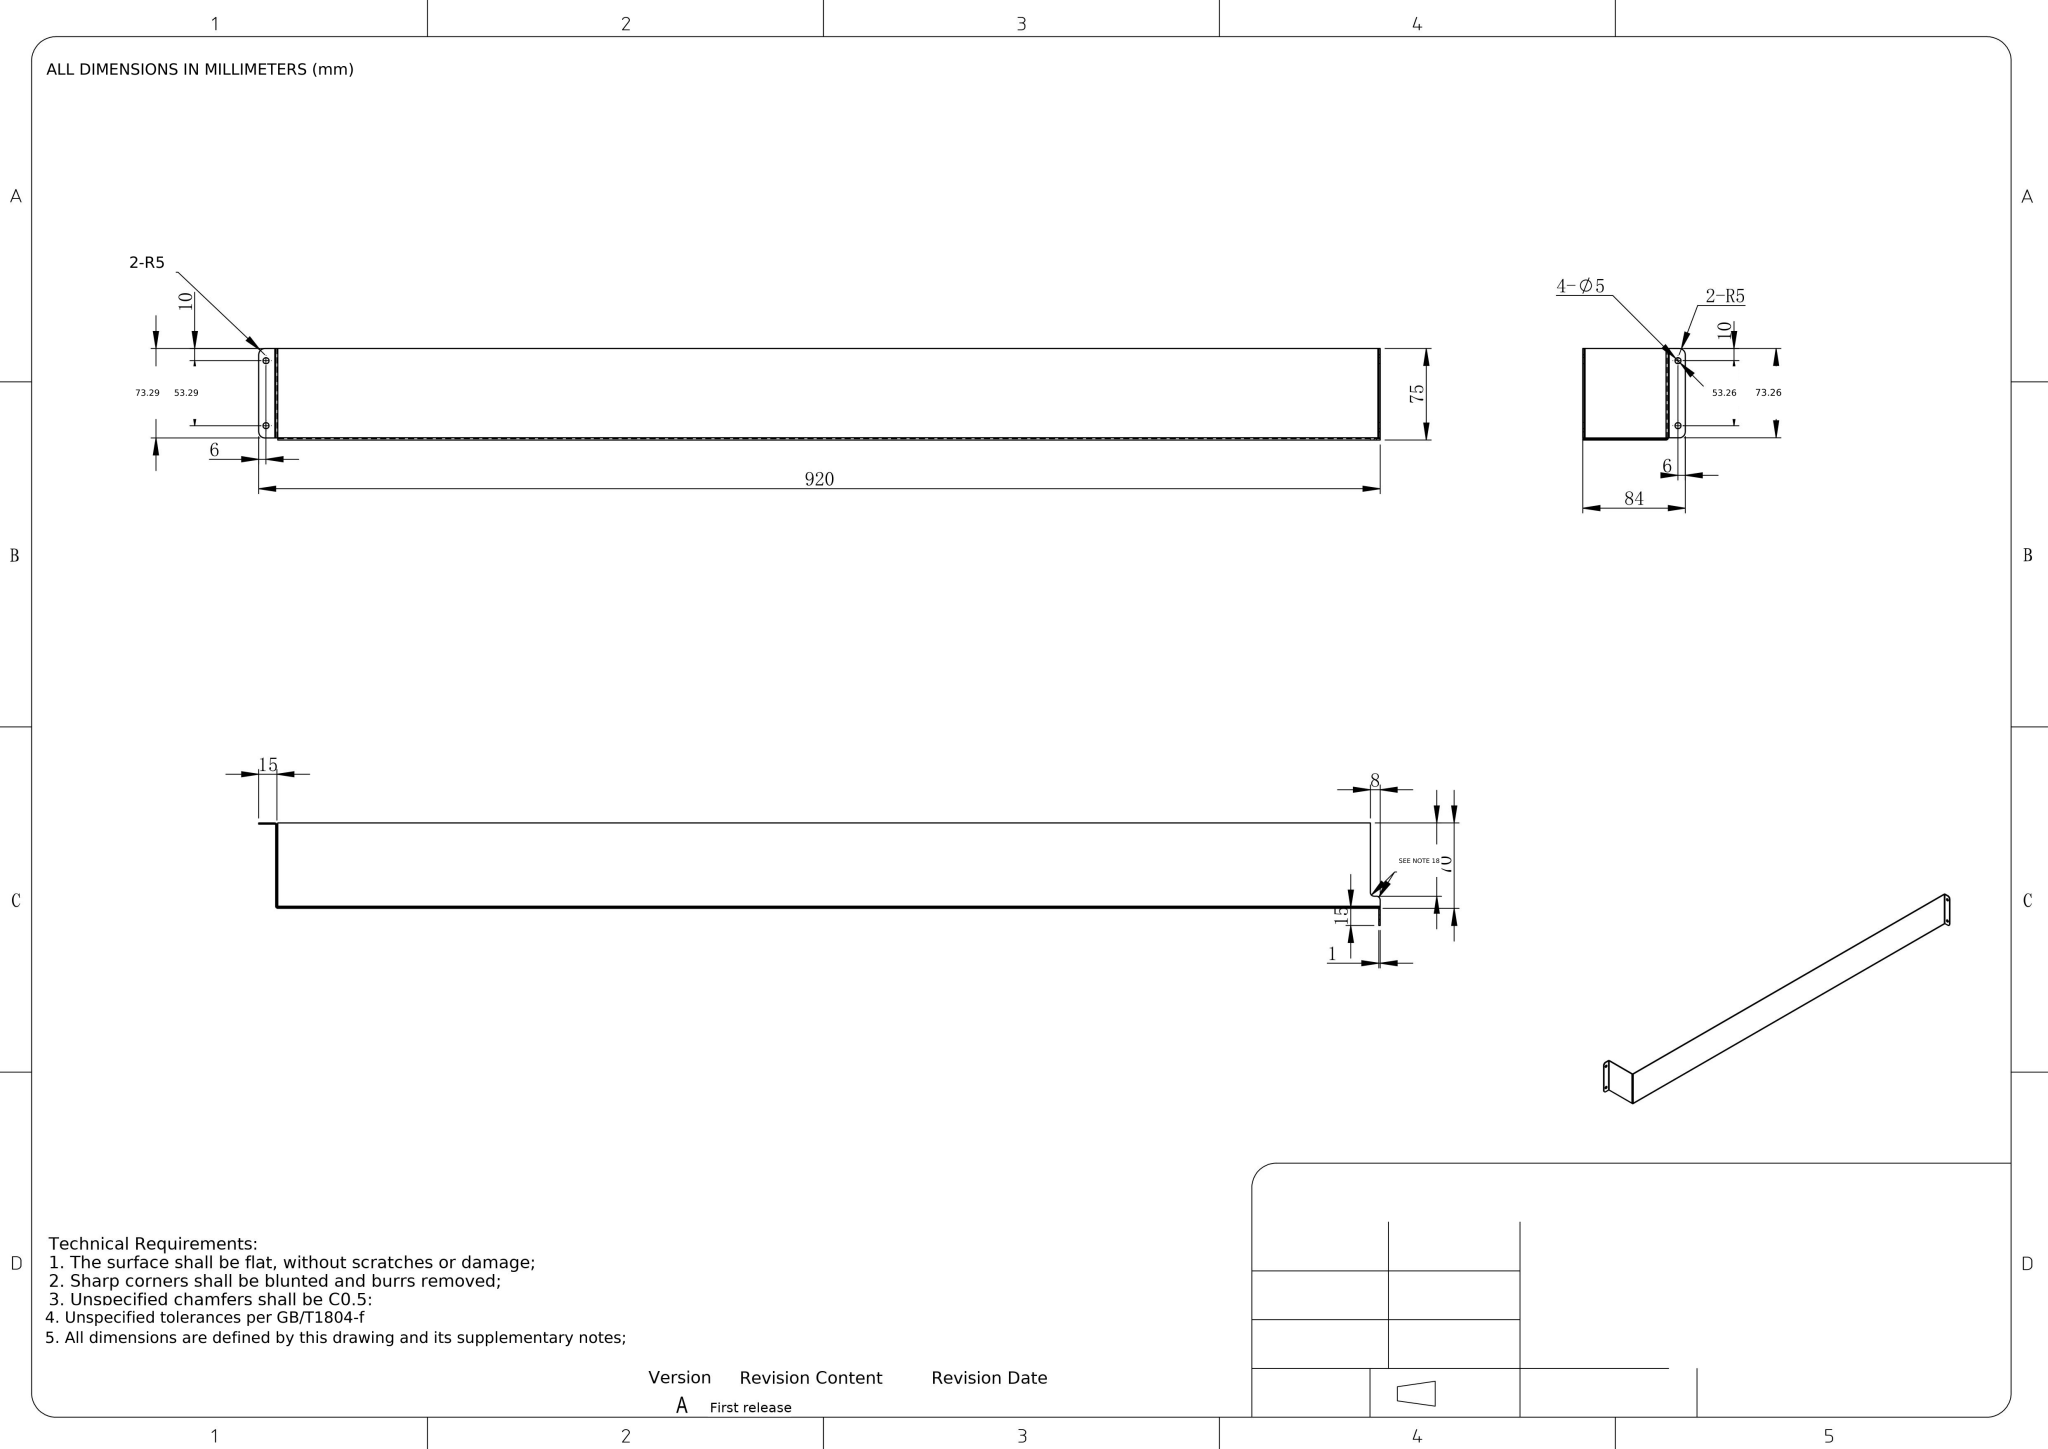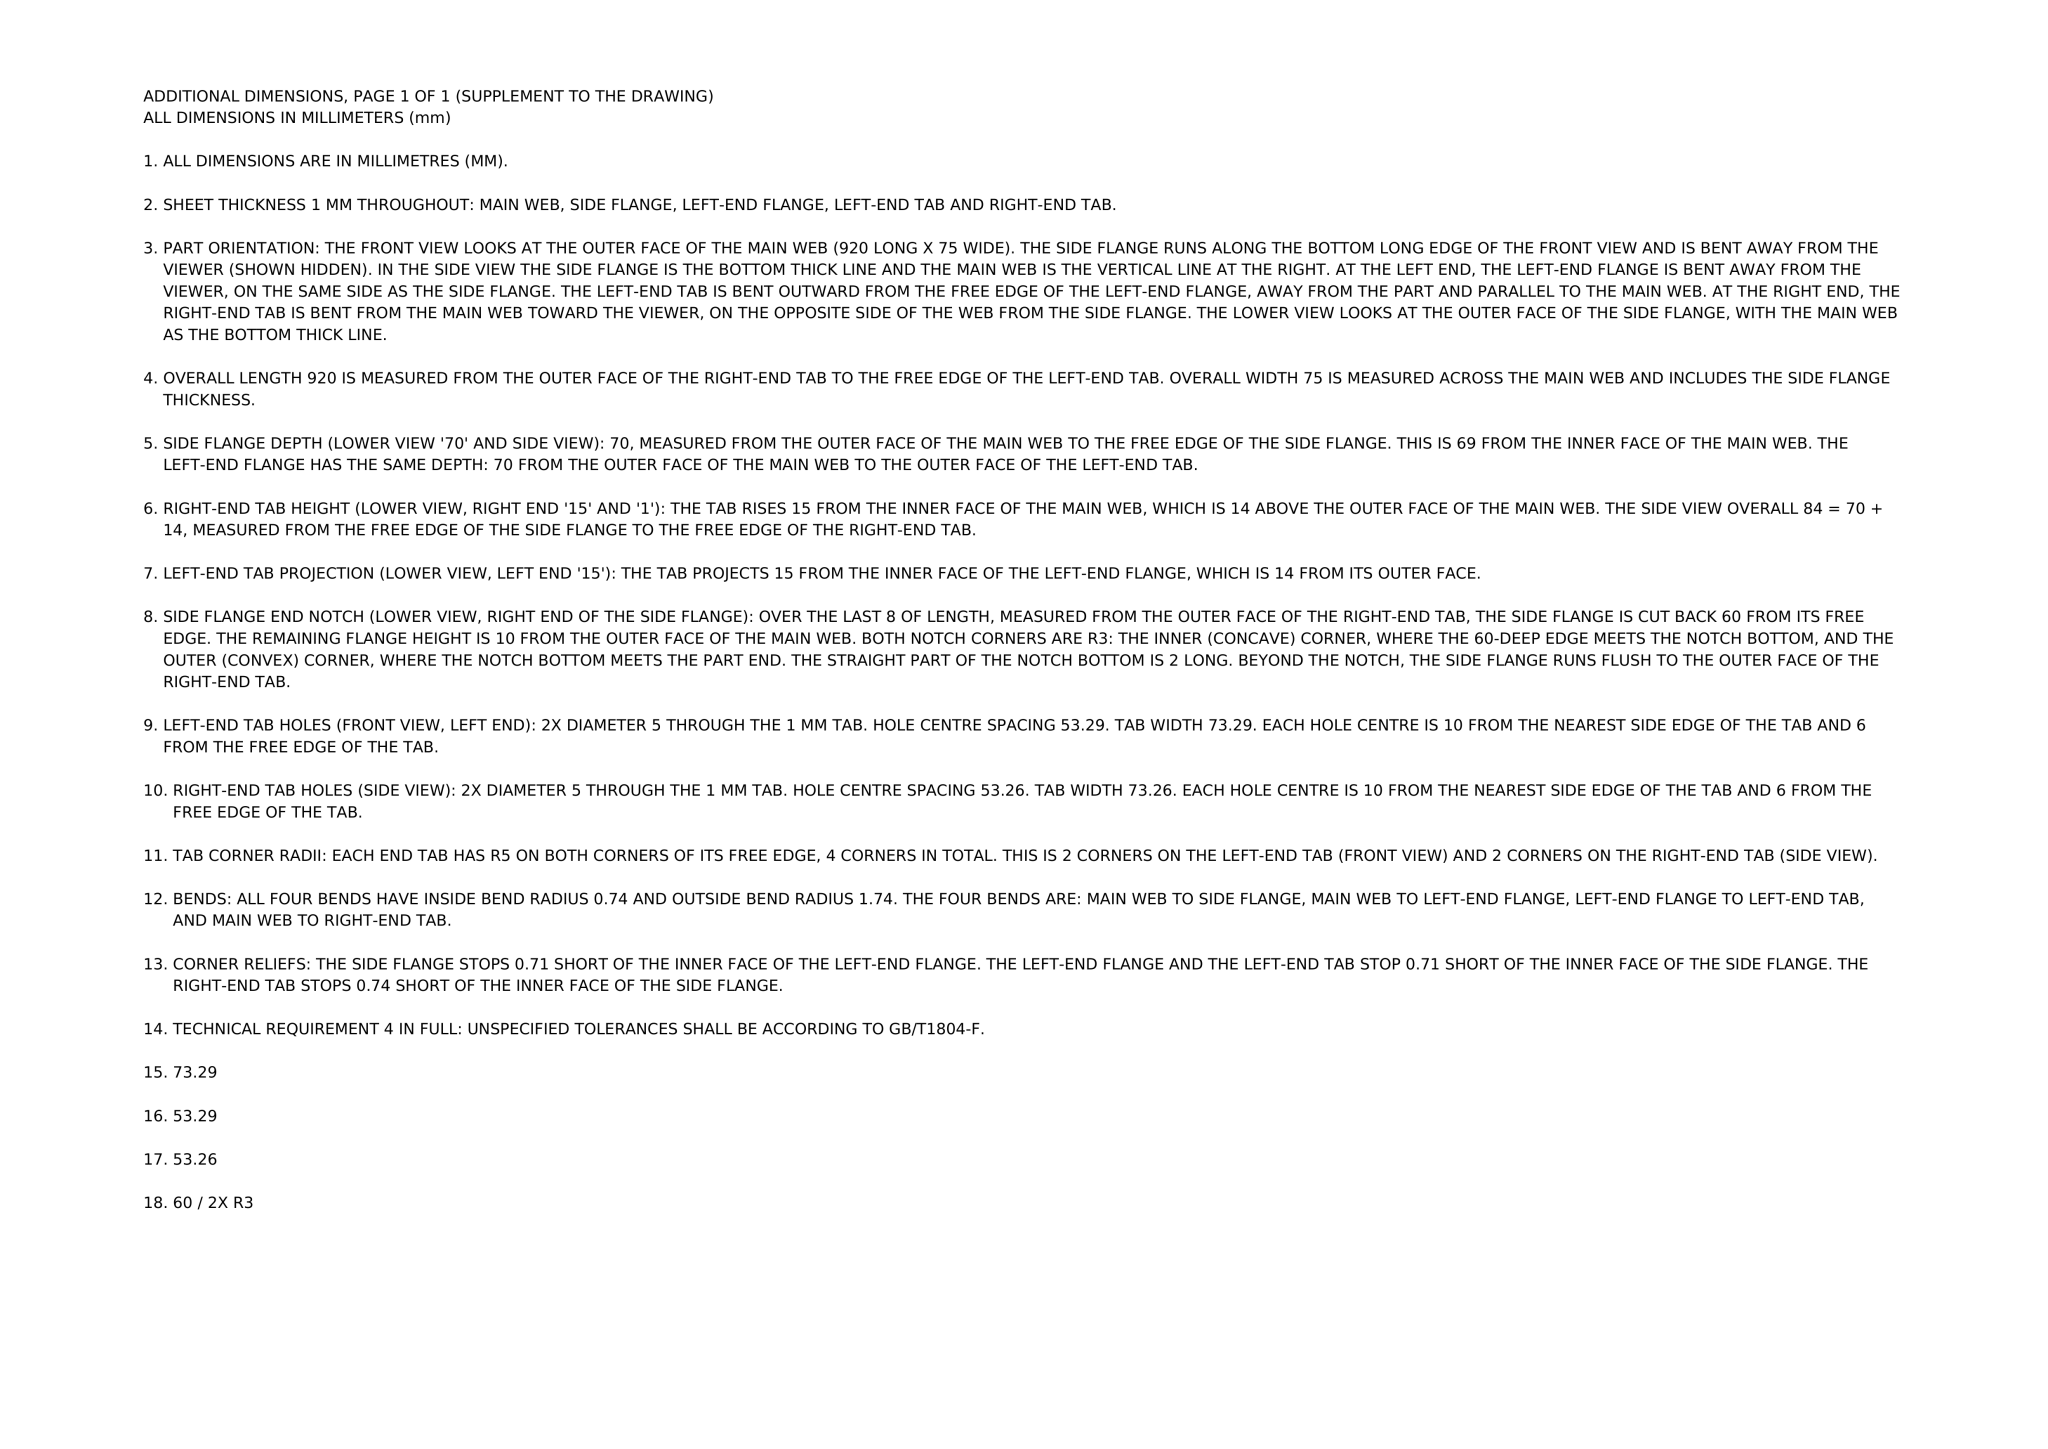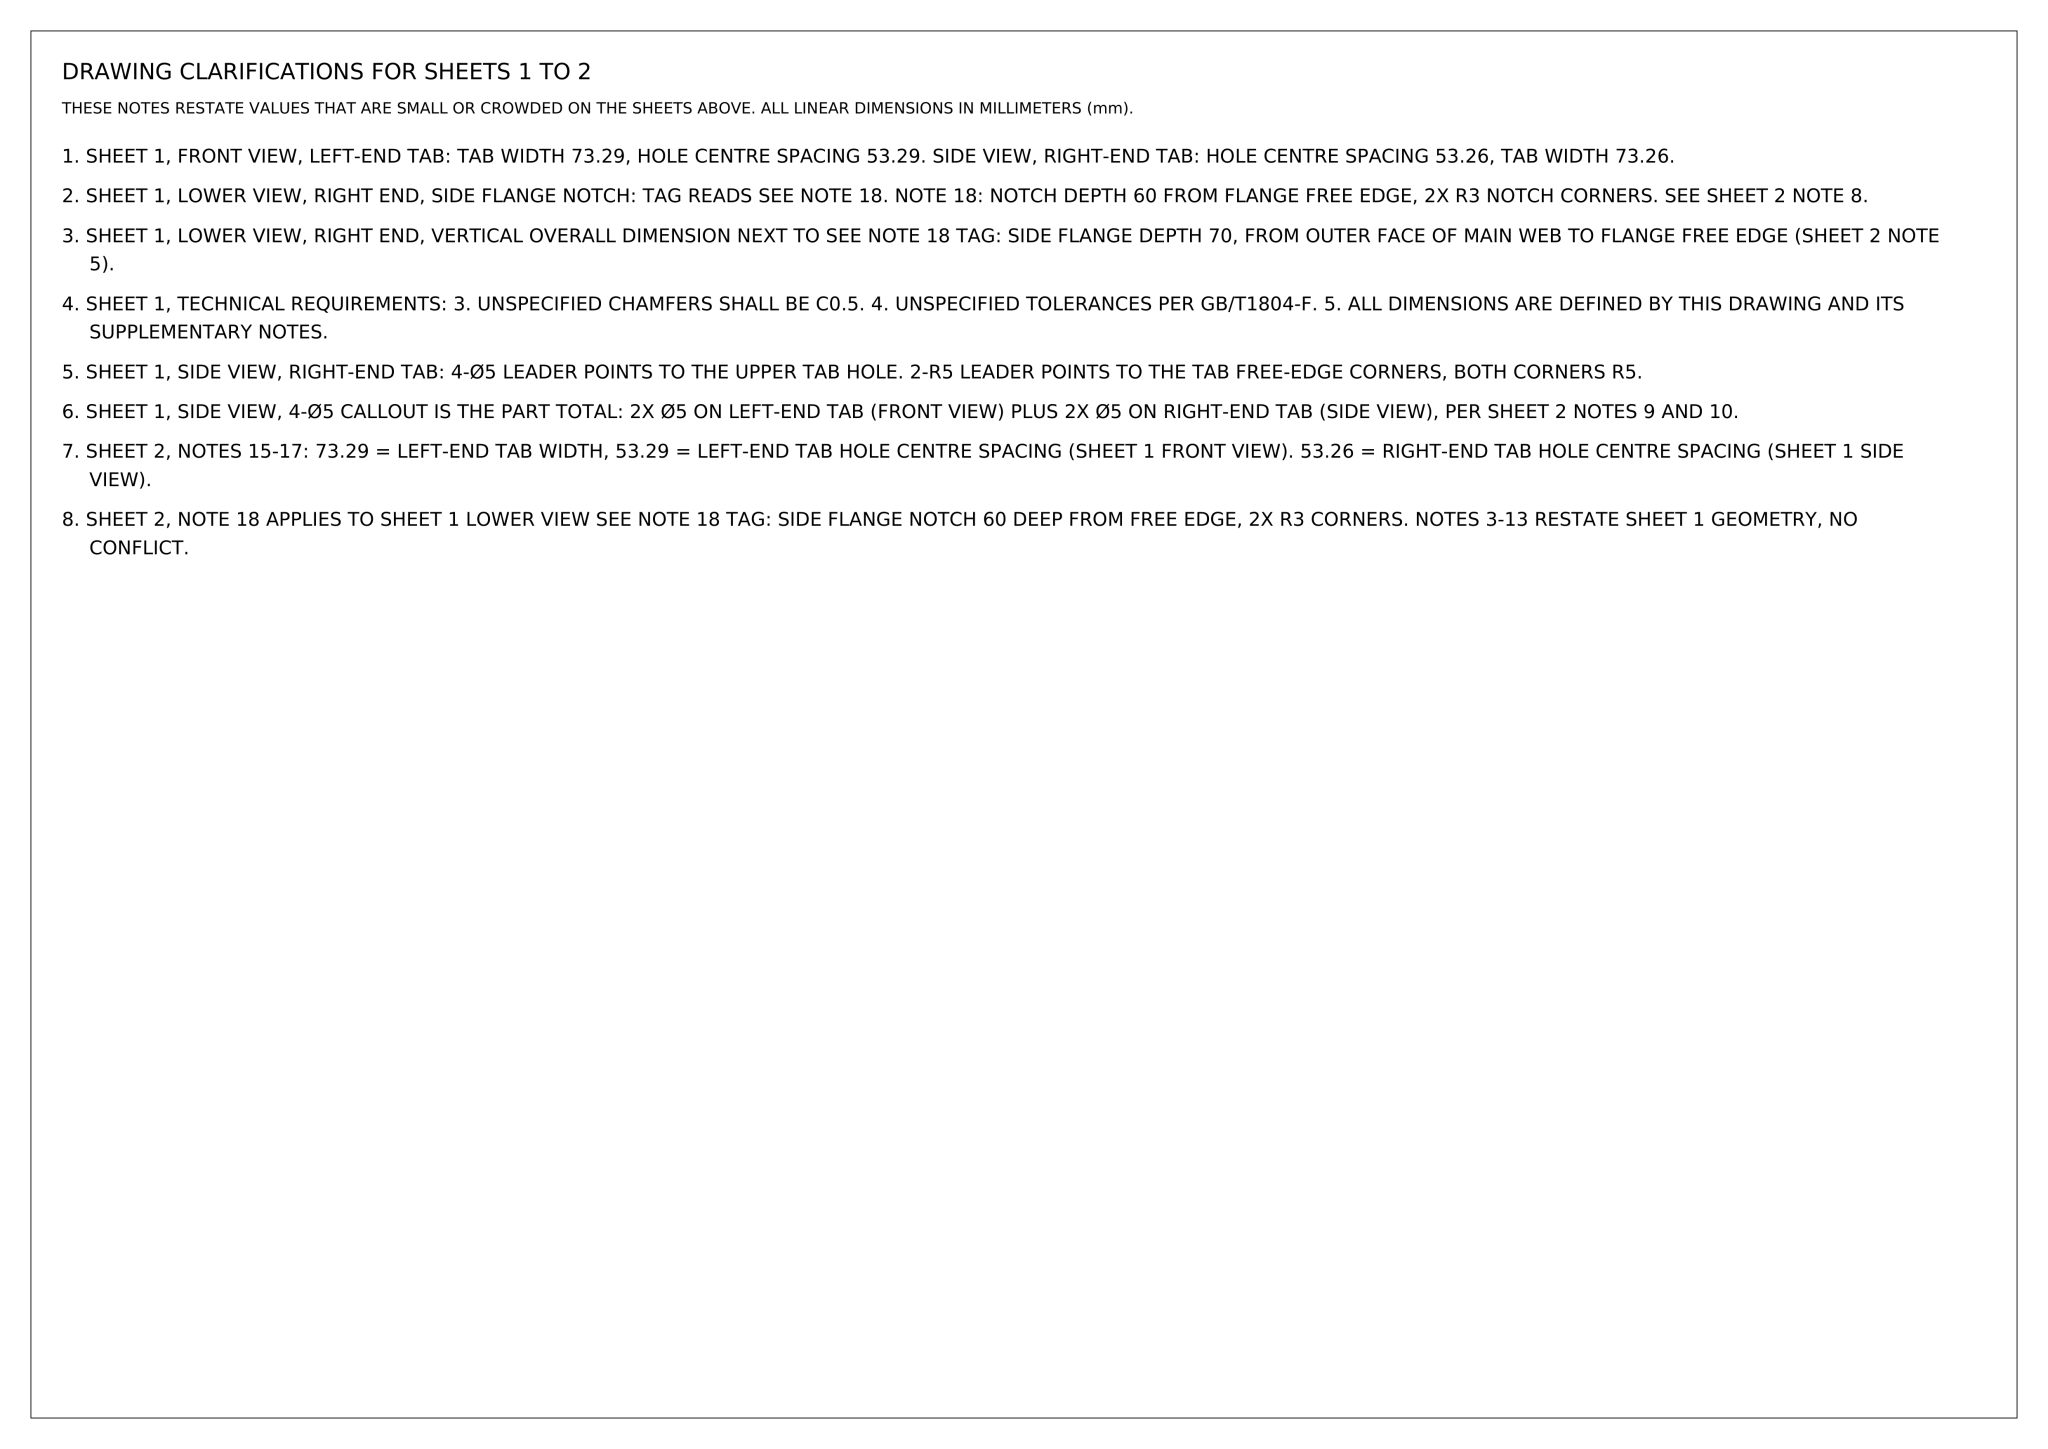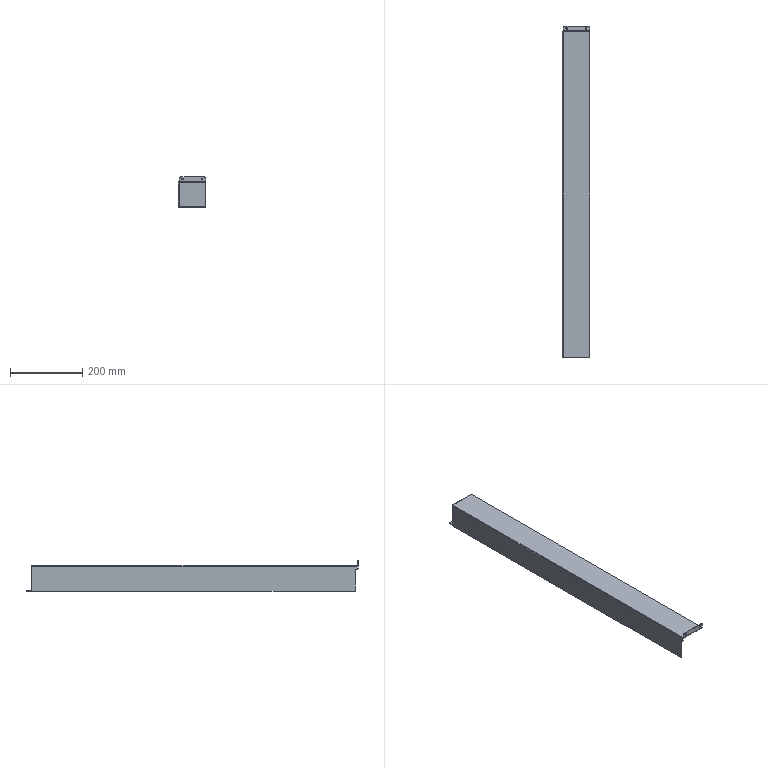Part | NX | mm | 1 solid | 55 faces | box 75 x 920 x 84 mm | volume 136276 mm3 | plane 31 | cylinder 22 | spline 2 | commonest cylinder face diameters 5 x8 3.473 x4 1.473 x4 10 x4 6 x2